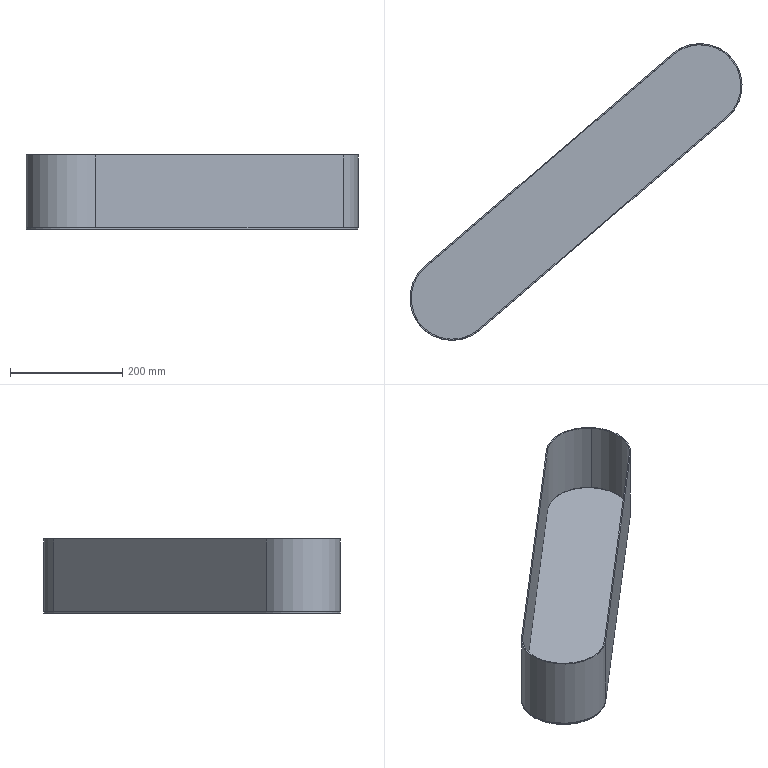Component | SolidWorks | BeltGuard-1 | 2 solids | 19 faces | box 591.77 x 528.9 x 132 mm | volume 633471 mm3 | plane 10 | cylinder 9 | commonest cylinder face diameters 150 x6 146 x3 | material Stainless Steel
build123d program:
from build123d import *

# Parameters (mm, degrees)
BOSS_EXTRUDE1_DEPTH = 2
BOSS_EXTRUDE2_DEPTH = 130


with BuildPart() as part:
    # Sketch1 → Boss-Extrude1 (new body)
    with BuildSketch(Plane.XY):
        with BuildLine():
            Line((0, 75), (582, 75))
            ThreePointArc((582, 75), (657, 0), (582, -75))
            Line((582, -75), (0, -75))
            ThreePointArc((0, -75), (-75, 0), (0, 75))
        make_face()
    extrude(amount=BOSS_EXTRUDE1_DEPTH)


with BuildPart() as body_2:
    # Sketch2 → Boss-Extrude2 (new body)
    with BuildSketch(Plane(origin=(0, 0, 0), x_dir=(-1, 0, 0), z_dir=(0, 0, -1))):
        with BuildLine():
            Line((0, 75), (-582, 75))
            ThreePointArc((-582, 75), (-657, 0), (-582, -75))
            Line((-582, -75), (0, -75))
            ThreePointArc((0, -75), (75, 0), (0, 75))
        make_face()
        with BuildLine():
            Line((0, 73), (-582, 73))
            ThreePointArc((-582, 73), (-655, 0), (-582, -73))
            Line((-582, -73), (0, -73))
            ThreePointArc((0, -73), (73, 0), (0, 73))
        make_face(mode=Mode.SUBTRACT)
    extrude(amount=BOSS_EXTRUDE2_DEPTH)


solid = Compound([part.part, body_2.part])

# Placed as in the assembly
solid = solid.moved(Location((-814.935, 937.863, -24.3), (180, 0, -40.619)))
STEP:
#1=COLOUR_RGB('',0.7922,0.8196,0.9333);
#2=FILL_AREA_STYLE_COLOUR('',#1);
#3=FILL_AREA_STYLE('',(#2));
#4=SURFACE_STYLE_FILL_AREA(#3);
#5=SURFACE_SIDE_STYLE('',(#4));
#6=SURFACE_STYLE_USAGE(.BOTH.,#5);
#7=PRESENTATION_STYLE_ASSIGNMENT((#6));
#8=CARTESIAN_POINT('',(-34.325,35.001,-1.035));
#9=VERTEX_POINT('',#8);
#10=CARTESIAN_POINT('',(-34.006,39.165,-1.035));
#11=VERTEX_POINT('',#10);
#12=CARTESIAN_POINT('',(-32.084,36.924,-1.035));
#13=DIRECTION('',(0.,0.,-1.));
#14=DIRECTION('',(0.7591,0.651,0.));
#15=AXIS2_PLACEMENT_3D('',#12,#13,#14);
#16=CIRCLE('',#15,2.953);
#17=EDGE_CURVE('',#9,#11,#16,.T.);
#18=ORIENTED_EDGE('',*,*,#17,.F.);
#19=CARTESIAN_POINT('',(-34.325,35.001,-0.9567));
#20=VERTEX_POINT('',#19);
#21=CARTESIAN_POINT('',(-34.325,35.001,-1.035));
#22=DIRECTION('',(-0.,-0.,1.));
#23=VECTOR('',#22,39.37);
#24=LINE('',#21,#23);
#25=EDGE_CURVE('',#9,#20,#24,.T.);
#26=ORIENTED_EDGE('',*,*,#25,.T.);
#27=CARTESIAN_POINT('',(-34.006,39.165,-0.9567));
#28=VERTEX_POINT('',#27);
#29=CARTESIAN_POINT('',(-32.084,36.924,-0.9567));
#30=DIRECTION('',(0.,0.,-1.));
#31=DIRECTION('',(0.7591,0.651,0.));
#32=AXIS2_PLACEMENT_3D('',#29,#30,#31);
#33=CIRCLE('',#32,2.953);
#34=EDGE_CURVE('',#20,#28,#33,.T.);
#35=ORIENTED_EDGE('',*,*,#34,.T.);
#36=CARTESIAN_POINT('',(-34.006,39.165,-1.035));
#37=DIRECTION('',(-0.,-0.,1.));
#38=VECTOR('',#37,39.37);
#39=LINE('',#36,#38);
#40=EDGE_CURVE('',#11,#28,#39,.T.);
#41=ORIENTED_EDGE('',*,*,#40,.F.);
#42=EDGE_LOOP('',(#18,#26,#35,#41));
#43=FACE_OUTER_BOUND('',#42,.T.);
#44=CARTESIAN_POINT('',(-32.084,36.924,-1.035));
#45=DIRECTION('',(-0.,-0.,1.));
#46=DIRECTION('',(-0.7591,-0.651,-0.));
#47=AXIS2_PLACEMENT_3D('',#44,#45,#46);
#48=CYLINDRICAL_SURFACE('',#47,2.953);
#49=ADVANCED_FACE('',(#43),#48,.T.);
#50=ORIENTED_EDGE('',*,*,#25,.F.);
#51=CARTESIAN_POINT('',(-30.162,34.682,-1.035));
#52=VERTEX_POINT('',#51);
#53=CARTESIAN_POINT('',(-32.084,36.924,-1.035));
#54=DIRECTION('',(0.,0.,-1.));
#55=DIRECTION('',(0.7591,0.651,0.));
#56=AXIS2_PLACEMENT_3D('',#53,#54,#55);
#57=CIRCLE('',#56,2.953);
#58=EDGE_CURVE('',#52,#9,#57,.T.);
#59=ORIENTED_EDGE('',*,*,#58,.F.);
#60=CARTESIAN_POINT('',(-30.162,34.682,-0.9567));
#61=VERTEX_POINT('',#60);
#62=CARTESIAN_POINT('',(-30.162,34.682,-1.035));
#63=DIRECTION('',(-0.,-0.,1.));
#64=VECTOR('',#63,39.37);
#65=LINE('',#62,#64);
#66=EDGE_CURVE('',#52,#61,#65,.T.);
#67=ORIENTED_EDGE('',*,*,#66,.T.);
#68=CARTESIAN_POINT('',(-32.084,36.924,-0.9567));
#69=DIRECTION('',(0.,0.,-1.));
#70=DIRECTION('',(0.7591,0.651,0.));
#71=AXIS2_PLACEMENT_3D('',#68,#69,#70);
#72=CIRCLE('',#71,2.953);
#73=EDGE_CURVE('',#61,#20,#72,.T.);
#74=ORIENTED_EDGE('',*,*,#73,.T.);
#75=EDGE_LOOP('',(#50,#59,#67,#74));
#76=FACE_OUTER_BOUND('',#75,.T.);
#77=CARTESIAN_POINT('',(-32.084,36.924,-1.035));
#78=DIRECTION('',(-0.,-0.,1.));
#79=DIRECTION('',(-0.7591,-0.651,-0.));
#80=AXIS2_PLACEMENT_3D('',#77,#78,#79);
#81=CYLINDRICAL_SURFACE('',#80,2.953);
#82=ADVANCED_FACE('',(#76),#81,.T.);
#83=CARTESIAN_POINT('',(-16.614,54.082,-0.9567));
#84=VERTEX_POINT('',#83);
#85=CARTESIAN_POINT('',(-34.006,39.165,-0.9567));
#86=DIRECTION('',(0.7591,0.651,0.));
#87=VECTOR('',#86,39.37);
#88=LINE('',#85,#87);
#89=EDGE_CURVE('',#28,#84,#88,.T.);
#90=ORIENTED_EDGE('',*,*,#89,.T.);
#91=CARTESIAN_POINT('',(-16.614,54.082,-1.035));
#92=VERTEX_POINT('',#91);
#93=CARTESIAN_POINT('',(-16.614,54.082,-1.035));
#94=DIRECTION('',(-0.,-0.,1.));
#95=VECTOR('',#94,39.37);
#96=LINE('',#93,#95);
#97=EDGE_CURVE('',#92,#84,#96,.T.);
#98=ORIENTED_EDGE('',*,*,#97,.F.);
#99=CARTESIAN_POINT('',(-34.006,39.165,-1.035));
#100=DIRECTION('',(0.7591,0.651,0.));
#101=VECTOR('',#100,39.37);
#102=LINE('',#99,#101);
#103=EDGE_CURVE('',#11,#92,#102,.T.);
#104=ORIENTED_EDGE('',*,*,#103,.F.);
#105=ORIENTED_EDGE('',*,*,#40,.T.);
#106=EDGE_LOOP('',(#90,#98,#104,#105));
#107=FACE_OUTER_BOUND('',#106,.T.);
#108=CARTESIAN_POINT('',(-34.006,39.165,-1.035));
#109=DIRECTION('',(0.651,-0.7591,-0.));
#110=DIRECTION('',(-0.7591,-0.651,-0.));
#111=AXIS2_PLACEMENT_3D('',#108,#109,#110);
#112=PLANE('',#111);
#113=ADVANCED_FACE('',(#107),#112,.F.);
#114=CARTESIAN_POINT('',(-12.769,49.6,-0.9567));
#115=VERTEX_POINT('',#114);
#116=CARTESIAN_POINT('',(-14.692,51.841,-0.9567));
#117=DIRECTION('',(0.,0.,-1.));
#118=DIRECTION('',(0.7591,0.651,0.));
#119=AXIS2_PLACEMENT_3D('',#116,#117,#118);
#120=CIRCLE('',#119,2.953);
#121=EDGE_CURVE('',#84,#115,#120,.T.);
#122=ORIENTED_EDGE('',*,*,#121,.T.);
#123=CARTESIAN_POINT('',(-12.769,49.6,-1.035));
#124=VERTEX_POINT('',#123);
#125=CARTESIAN_POINT('',(-12.769,49.6,-1.035));
#126=DIRECTION('',(-0.,-0.,1.));
#127=VECTOR('',#126,39.37);
#128=LINE('',#125,#127);
#129=EDGE_CURVE('',#124,#115,#128,.T.);
#130=ORIENTED_EDGE('',*,*,#129,.F.);
#131=CARTESIAN_POINT('',(-14.692,51.841,-1.035));
#132=DIRECTION('',(0.,0.,-1.));
#133=DIRECTION('',(0.7591,0.651,0.));
#134=AXIS2_PLACEMENT_3D('',#131,#132,#133);
#135=CIRCLE('',#134,2.953);
#136=EDGE_CURVE('',#92,#124,#135,.T.);
#137=ORIENTED_EDGE('',*,*,#136,.F.);
#138=ORIENTED_EDGE('',*,*,#97,.T.);
#139=EDGE_LOOP('',(#122,#130,#137,#138));
#140=FACE_OUTER_BOUND('',#139,.T.);
#141=CARTESIAN_POINT('',(-14.692,51.841,-1.035));
#142=DIRECTION('',(-0.,-0.,1.));
#143=DIRECTION('',(-0.7591,-0.651,-0.));
#144=AXIS2_PLACEMENT_3D('',#141,#142,#143);
#145=CYLINDRICAL_SURFACE('',#144,2.953);
#146=ADVANCED_FACE('',(#140),#145,.T.);
#147=CARTESIAN_POINT('',(-30.162,34.682,-0.9567));
#148=DIRECTION('',(-0.7591,-0.651,-0.));
#149=VECTOR('',#148,39.37);
#150=LINE('',#147,#149);
#151=EDGE_CURVE('',#115,#61,#150,.T.);
#152=ORIENTED_EDGE('',*,*,#151,.T.);
#153=ORIENTED_EDGE('',*,*,#66,.F.);
#154=CARTESIAN_POINT('',(-30.162,34.682,-1.035));
#155=DIRECTION('',(-0.7591,-0.651,-0.));
#156=VECTOR('',#155,39.37);
#157=LINE('',#154,#156);
#158=EDGE_CURVE('',#124,#52,#157,.T.);
#159=ORIENTED_EDGE('',*,*,#158,.F.);
#160=ORIENTED_EDGE('',*,*,#129,.T.);
#161=EDGE_LOOP('',(#152,#153,#159,#160));
#162=FACE_OUTER_BOUND('',#161,.T.);
#163=CARTESIAN_POINT('',(-30.162,34.682,-1.035));
#164=DIRECTION('',(-0.651,0.7591,0.));
#165=DIRECTION('',(0.7591,0.651,0.));
#166=AXIS2_PLACEMENT_3D('',#163,#164,#165);
#167=PLANE('',#166);
#168=ADVANCED_FACE('',(#162),#167,.F.);
#169=ORIENTED_EDGE('',*,*,#58,.T.);
#170=ORIENTED_EDGE('',*,*,#17,.T.);
#171=ORIENTED_EDGE('',*,*,#103,.T.);
#172=ORIENTED_EDGE('',*,*,#136,.T.);
#173=ORIENTED_EDGE('',*,*,#158,.T.);
#174=EDGE_LOOP('',(#169,#170,#171,#172,#173));
#175=FACE_OUTER_BOUND('',#174,.T.);
#176=CARTESIAN_POINT('',(-32.084,36.924,-1.035));
#177=DIRECTION('',(0.,0.,-1.));
#178=DIRECTION('',(0.7591,0.651,0.));
#179=AXIS2_PLACEMENT_3D('',#176,#177,#178);
#180=PLANE('',#179);
#181=ADVANCED_FACE('',(#175),#180,.T.);
#182=ORIENTED_EDGE('',*,*,#73,.F.);
#183=ORIENTED_EDGE('',*,*,#151,.F.);
#184=ORIENTED_EDGE('',*,*,#121,.F.);
#185=ORIENTED_EDGE('',*,*,#89,.F.);
#186=ORIENTED_EDGE('',*,*,#34,.F.);
#187=EDGE_LOOP('',(#182,#183,#184,#185,#186));
#188=FACE_OUTER_BOUND('',#187,.T.);
#189=CARTESIAN_POINT('',(-32.084,36.924,-0.9567));
#190=DIRECTION('',(0.,0.,-1.));
#191=DIRECTION('',(0.7591,0.651,0.));
#192=AXIS2_PLACEMENT_3D('',#189,#190,#191);
#193=PLANE('',#192);
#194=ADVANCED_FACE('',(#188),#193,.F.);
#195=CLOSED_SHELL('',(#49,#82,#113,#146,#168,#181,#194));
#196=MANIFOLD_SOLID_BREP('',#195);
#197=STYLED_ITEM('',(#7),#196);
#198=PRESENTATION_LAYER_ASSIGNMENT('','',(#197));
#199=CARTESIAN_POINT('',(-12.82,49.659,4.161));
#200=VERTEX_POINT('',#199);
#201=CARTESIAN_POINT('',(-12.51,53.712,4.161));
#202=VERTEX_POINT('',#201);
#203=CARTESIAN_POINT('',(-14.692,51.841,4.161));
#204=DIRECTION('',(-0.,-0.,1.));
#205=DIRECTION('',(-0.7591,-0.651,-0.));
#206=AXIS2_PLACEMENT_3D('',#203,#204,#205);
#207=CIRCLE('',#206,2.874);
#208=EDGE_CURVE('',#200,#202,#207,.T.);
#209=ORIENTED_EDGE('',*,*,#208,.T.);
#210=CARTESIAN_POINT('',(-12.51,53.712,-0.9567));
#211=VERTEX_POINT('',#210);
#212=CARTESIAN_POINT('',(-12.51,53.712,4.161));
#213=DIRECTION('',(0.,0.,-1.));
#214=VECTOR('',#213,39.37);
#215=LINE('',#212,#214);
#216=EDGE_CURVE('',#202,#211,#215,.T.);
#217=ORIENTED_EDGE('',*,*,#216,.T.);
#218=CARTESIAN_POINT('',(-12.82,49.659,-0.9567));
#219=VERTEX_POINT('',#218);
#220=CARTESIAN_POINT('',(-14.692,51.841,-0.9567));
#221=DIRECTION('',(-0.,-0.,1.));
#222=DIRECTION('',(-0.7591,-0.651,-0.));
#223=AXIS2_PLACEMENT_3D('',#220,#221,#222);
#224=CIRCLE('',#223,2.874);
#225=EDGE_CURVE('',#219,#211,#224,.T.);
#226=ORIENTED_EDGE('',*,*,#225,.F.);
#227=CARTESIAN_POINT('',(-12.82,49.659,4.161));
#228=DIRECTION('',(0.,0.,-1.));
#229=VECTOR('',#228,39.37);
#230=LINE('',#227,#229);
#231=EDGE_CURVE('',#200,#219,#230,.T.);
#232=ORIENTED_EDGE('',*,*,#231,.F.);
#233=EDGE_LOOP('',(#209,#217,#226,#232));
#234=FACE_OUTER_BOUND('',#233,.T.);
#235=CARTESIAN_POINT('',(-14.692,51.841,4.161));
#236=DIRECTION('',(0.,0.,-1.));
#237=DIRECTION('',(0.7591,0.651,0.));
#238=AXIS2_PLACEMENT_3D('',#235,#236,#237);
#239=CYLINDRICAL_SURFACE('',#238,2.874);
#240=ADVANCED_FACE('',(#234),#239,.F.);
#241=CARTESIAN_POINT('',(-12.45,53.763,4.161));
#242=VERTEX_POINT('',#241);
#243=CARTESIAN_POINT('',(-16.614,54.082,4.161));
#244=VERTEX_POINT('',#243);
#245=CARTESIAN_POINT('',(-14.692,51.841,4.161));
#246=DIRECTION('',(-0.,-0.,1.));
#247=DIRECTION('',(-0.7591,-0.651,-0.));
#248=AXIS2_PLACEMENT_3D('',#245,#246,#247);
#249=CIRCLE('',#248,2.953);
#250=EDGE_CURVE('',#242,#244,#249,.T.);
#251=ORIENTED_EDGE('',*,*,#250,.F.);
#252=CARTESIAN_POINT('',(-12.45,53.763,-0.9567));
#253=VERTEX_POINT('',#252);
#254=CARTESIAN_POINT('',(-12.45,53.763,4.161));
#255=DIRECTION('',(0.,0.,-1.));
#256=VECTOR('',#255,39.37);
#257=LINE('',#254,#256);
#258=EDGE_CURVE('',#242,#253,#257,.T.);
#259=ORIENTED_EDGE('',*,*,#258,.T.);
#260=CARTESIAN_POINT('',(-16.614,54.082,-0.9567));
#261=VERTEX_POINT('',#260);
#262=CARTESIAN_POINT('',(-14.692,51.841,-0.9567));
#263=DIRECTION('',(-0.,-0.,1.));
#264=DIRECTION('',(-0.7591,-0.651,-0.));
#265=AXIS2_PLACEMENT_3D('',#262,#263,#264);
#266=CIRCLE('',#265,2.953);
#267=EDGE_CURVE('',#253,#261,#266,.T.);
#268=ORIENTED_EDGE('',*,*,#267,.T.);
#269=CARTESIAN_POINT('',(-16.614,54.082,4.161));
#270=DIRECTION('',(0.,0.,-1.));
#271=VECTOR('',#270,39.37);
#272=LINE('',#269,#271);
#273=EDGE_CURVE('',#244,#261,#272,.T.);
#274=ORIENTED_EDGE('',*,*,#273,.F.);
#275=EDGE_LOOP('',(#251,#259,#268,#274));
#276=FACE_OUTER_BOUND('',#275,.T.);
#277=CARTESIAN_POINT('',(-14.692,51.841,4.161));
#278=DIRECTION('',(0.,0.,-1.));
#279=DIRECTION('',(0.7591,0.651,0.));
#280=AXIS2_PLACEMENT_3D('',#277,#278,#279);
#281=CYLINDRICAL_SURFACE('',#280,2.953);
#282=ADVANCED_FACE('',(#276),#281,.T.);
#283=CARTESIAN_POINT('',(-34.006,39.165,4.161));
#284=VERTEX_POINT('',#283);
#285=CARTESIAN_POINT('',(-30.162,34.682,4.161));
#286=VERTEX_POINT('',#285);
#287=CARTESIAN_POINT('',(-32.084,36.924,4.161));
#288=DIRECTION('',(-0.,-0.,1.));
#289=DIRECTION('',(-0.7591,-0.651,-0.));
#290=AXIS2_PLACEMENT_3D('',#287,#288,#289);
#291=CIRCLE('',#290,2.953);
#292=EDGE_CURVE('',#284,#286,#291,.T.);
#293=ORIENTED_EDGE('',*,*,#292,.T.);
#294=CARTESIAN_POINT('',(-12.769,49.6,4.161));
#295=VERTEX_POINT('',#294);
#296=CARTESIAN_POINT('',(-30.162,34.682,4.161));
#297=DIRECTION('',(0.7591,0.651,0.));
#298=VECTOR('',#297,39.37);
#299=LINE('',#296,#298);
#300=EDGE_CURVE('',#286,#295,#299,.T.);
#301=ORIENTED_EDGE('',*,*,#300,.T.);
#302=CARTESIAN_POINT('',(-14.692,51.841,4.161));
#303=DIRECTION('',(-0.,-0.,1.));
#304=DIRECTION('',(-0.7591,-0.651,-0.));
#305=AXIS2_PLACEMENT_3D('',#302,#303,#304);
#306=CIRCLE('',#305,2.953);
#307=EDGE_CURVE('',#295,#242,#306,.T.);
#308=ORIENTED_EDGE('',*,*,#307,.T.);
#309=ORIENTED_EDGE('',*,*,#250,.T.);
#310=CARTESIAN_POINT('',(-16.614,54.082,4.161));
#311=DIRECTION('',(-0.7591,-0.651,-0.));
#312=VECTOR('',#311,39.37);
#313=LINE('',#310,#312);
#314=EDGE_CURVE('',#244,#284,#313,.T.);
#315=ORIENTED_EDGE('',*,*,#314,.T.);
#316=EDGE_LOOP('',(#293,#301,#308,#309,#315));
#317=FACE_OUTER_BOUND('',#316,.T.);
#318=CARTESIAN_POINT('',(-30.213,34.742,4.161));
#319=VERTEX_POINT('',#318);
#320=CARTESIAN_POINT('',(-30.213,34.742,4.161));
#321=DIRECTION('',(0.7591,0.651,0.));
#322=VECTOR('',#321,39.37);
#323=LINE('',#320,#322);
#324=EDGE_CURVE('',#319,#200,#323,.T.);
#325=ORIENTED_EDGE('',*,*,#324,.F.);
#326=CARTESIAN_POINT('',(-33.955,39.105,4.161));
#327=VERTEX_POINT('',#326);
#328=CARTESIAN_POINT('',(-32.084,36.924,4.161));
#329=DIRECTION('',(-0.,-0.,1.));
#330=DIRECTION('',(-0.7591,-0.651,-0.));
#331=AXIS2_PLACEMENT_3D('',#328,#329,#330);
#332=CIRCLE('',#331,2.874);
#333=EDGE_CURVE('',#327,#319,#332,.T.);
#334=ORIENTED_EDGE('',*,*,#333,.F.);
#335=CARTESIAN_POINT('',(-16.563,54.023,4.161));
#336=VERTEX_POINT('',#335);
#337=CARTESIAN_POINT('',(-16.563,54.023,4.161));
#338=DIRECTION('',(-0.7591,-0.651,-0.));
#339=VECTOR('',#338,39.37);
#340=LINE('',#337,#339);
#341=EDGE_CURVE('',#336,#327,#340,.T.);
#342=ORIENTED_EDGE('',*,*,#341,.F.);
#343=CARTESIAN_POINT('',(-14.692,51.841,4.161));
#344=DIRECTION('',(-0.,-0.,1.));
#345=DIRECTION('',(-0.7591,-0.651,-0.));
#346=AXIS2_PLACEMENT_3D('',#343,#344,#345);
#347=CIRCLE('',#346,2.874);
#348=EDGE_CURVE('',#202,#336,#347,.T.);
#349=ORIENTED_EDGE('',*,*,#348,.F.);
#350=ORIENTED_EDGE('',*,*,#208,.F.);
#351=EDGE_LOOP('',(#325,#334,#342,#349,#350));
#352=FACE_BOUND('',#351,.T.);
#353=CARTESIAN_POINT('',(-32.084,36.924,4.161));
#354=DIRECTION('',(-0.,-0.,1.));
#355=DIRECTION('',(-0.7591,-0.651,-0.));
#356=AXIS2_PLACEMENT_3D('',#353,#354,#355);
#357=PLANE('',#356);
#358=ADVANCED_FACE('',(#317,#352),#357,.T.);
#359=CARTESIAN_POINT('',(-34.006,39.165,-0.9567));
#360=VERTEX_POINT('',#359);
#361=CARTESIAN_POINT('',(-30.162,34.682,-0.9567));
#362=VERTEX_POINT('',#361);
#363=CARTESIAN_POINT('',(-32.084,36.924,-0.9567));
#364=DIRECTION('',(-0.,-0.,1.));
#365=DIRECTION('',(-0.7591,-0.651,-0.));
#366=AXIS2_PLACEMENT_3D('',#363,#364,#365);
#367=CIRCLE('',#366,2.953);
#368=EDGE_CURVE('',#360,#362,#367,.T.);
#369=ORIENTED_EDGE('',*,*,#368,.F.);
#370=CARTESIAN_POINT('',(-16.614,54.082,-0.9567));
#371=DIRECTION('',(-0.7591,-0.651,-0.));
#372=VECTOR('',#371,39.37);
#373=LINE('',#370,#372);
#374=EDGE_CURVE('',#261,#360,#373,.T.);
#375=ORIENTED_EDGE('',*,*,#374,.F.);
#376=ORIENTED_EDGE('',*,*,#267,.F.);
#377=CARTESIAN_POINT('',(-12.769,49.6,-0.9567));
#378=VERTEX_POINT('',#377);
#379=CARTESIAN_POINT('',(-14.692,51.841,-0.9567));
#380=DIRECTION('',(-0.,-0.,1.));
#381=DIRECTION('',(-0.7591,-0.651,-0.));
#382=AXIS2_PLACEMENT_3D('',#379,#380,#381);
#383=CIRCLE('',#382,2.953);
#384=EDGE_CURVE('',#378,#253,#383,.T.);
#385=ORIENTED_EDGE('',*,*,#384,.F.);
#386=CARTESIAN_POINT('',(-30.162,34.682,-0.9567));
#387=DIRECTION('',(0.7591,0.651,0.));
#388=VECTOR('',#387,39.37);
#389=LINE('',#386,#388);
#390=EDGE_CURVE('',#362,#378,#389,.T.);
#391=ORIENTED_EDGE('',*,*,#390,.F.);
#392=EDGE_LOOP('',(#369,#375,#376,#385,#391));
#393=FACE_OUTER_BOUND('',#392,.T.);
#394=CARTESIAN_POINT('',(-33.955,39.105,-0.9567));
#395=VERTEX_POINT('',#394);
#396=CARTESIAN_POINT('',(-30.213,34.742,-0.9567));
#397=VERTEX_POINT('',#396);
#398=CARTESIAN_POINT('',(-32.084,36.924,-0.9567));
#399=DIRECTION('',(-0.,-0.,1.));
#400=DIRECTION('',(-0.7591,-0.651,-0.));
#401=AXIS2_PLACEMENT_3D('',#398,#399,#400);
#402=CIRCLE('',#401,2.874);
#403=EDGE_CURVE('',#395,#397,#402,.T.);
#404=ORIENTED_EDGE('',*,*,#403,.T.);
#405=CARTESIAN_POINT('',(-30.213,34.742,-0.9567));
#406=DIRECTION('',(0.7591,0.651,0.));
#407=VECTOR('',#406,39.37);
#408=LINE('',#405,#407);
#409=EDGE_CURVE('',#397,#219,#408,.T.);
#410=ORIENTED_EDGE('',*,*,#409,.T.);
#411=ORIENTED_EDGE('',*,*,#225,.T.);
#412=CARTESIAN_POINT('',(-16.563,54.023,-0.9567));
#413=VERTEX_POINT('',#412);
#414=CARTESIAN_POINT('',(-14.692,51.841,-0.9567));
#415=DIRECTION('',(-0.,-0.,1.));
#416=DIRECTION('',(-0.7591,-0.651,-0.));
#417=AXIS2_PLACEMENT_3D('',#414,#415,#416);
#418=CIRCLE('',#417,2.874);
#419=EDGE_CURVE('',#211,#413,#418,.T.);
#420=ORIENTED_EDGE('',*,*,#419,.T.);
#421=CARTESIAN_POINT('',(-16.563,54.023,-0.9567));
#422=DIRECTION('',(-0.7591,-0.651,-0.));
#423=VECTOR('',#422,39.37);
#424=LINE('',#421,#423);
#425=EDGE_CURVE('',#413,#395,#424,.T.);
#426=ORIENTED_EDGE('',*,*,#425,.T.);
#427=EDGE_LOOP('',(#404,#410,#411,#420,#426));
#428=FACE_BOUND('',#427,.T.);
#429=CARTESIAN_POINT('',(-32.084,36.924,-0.9567));
#430=DIRECTION('',(-0.,-0.,1.));
#431=DIRECTION('',(-0.7591,-0.651,-0.));
#432=AXIS2_PLACEMENT_3D('',#429,#430,#431);
#433=PLANE('',#432);
#434=ADVANCED_FACE('',(#393,#428),#433,.F.);
#435=ORIENTED_EDGE('',*,*,#368,.T.);
#436=CARTESIAN_POINT('',(-30.162,34.682,4.161));
#437=DIRECTION('',(0.,0.,-1.));
#438=VECTOR('',#437,39.37);
#439=LINE('',#436,#438);
#440=EDGE_CURVE('',#286,#362,#439,.T.);
#441=ORIENTED_EDGE('',*,*,#440,.F.);
#442=ORIENTED_EDGE('',*,*,#292,.F.);
#443=CARTESIAN_POINT('',(-34.006,39.165,4.161));
#444=DIRECTION('',(0.,0.,-1.));
#445=VECTOR('',#444,39.37);
#446=LINE('',#443,#445);
#447=EDGE_CURVE('',#284,#360,#446,.T.);
#448=ORIENTED_EDGE('',*,*,#447,.T.);
#449=EDGE_LOOP('',(#435,#441,#442,#448));
#450=FACE_OUTER_BOUND('',#449,.T.);
#451=CARTESIAN_POINT('',(-32.084,36.924,4.161));
#452=DIRECTION('',(0.,0.,-1.));
#453=DIRECTION('',(0.7591,0.651,0.));
#454=AXIS2_PLACEMENT_3D('',#451,#452,#453);
#455=CYLINDRICAL_SURFACE('',#454,2.953);
#456=ADVANCED_FACE('',(#450),#455,.T.);
#457=ORIENTED_EDGE('',*,*,#390,.T.);
#458=CARTESIAN_POINT('',(-12.769,49.6,4.161));
#459=DIRECTION('',(0.,0.,-1.));
#460=VECTOR('',#459,39.37);
#461=LINE('',#458,#460);
#462=EDGE_CURVE('',#295,#378,#461,.T.);
#463=ORIENTED_EDGE('',*,*,#462,.F.);
#464=ORIENTED_EDGE('',*,*,#300,.F.);
#465=ORIENTED_EDGE('',*,*,#440,.T.);
#466=EDGE_LOOP('',(#457,#463,#464,#465));
#467=FACE_OUTER_BOUND('',#466,.T.);
#468=CARTESIAN_POINT('',(-30.162,34.682,4.161));
#469=DIRECTION('',(-0.651,0.7591,0.));
#470=DIRECTION('',(0.7591,0.651,0.));
#471=AXIS2_PLACEMENT_3D('',#468,#469,#470);
#472=PLANE('',#471);
#473=ADVANCED_FACE('',(#467),#472,.F.);
#474=ORIENTED_EDGE('',*,*,#258,.F.);
#475=ORIENTED_EDGE('',*,*,#307,.F.);
#476=ORIENTED_EDGE('',*,*,#462,.T.);
#477=ORIENTED_EDGE('',*,*,#384,.T.);
#478=EDGE_LOOP('',(#474,#475,#476,#477));
#479=FACE_OUTER_BOUND('',#478,.T.);
#480=CARTESIAN_POINT('',(-14.692,51.841,4.161));
#481=DIRECTION('',(0.,0.,-1.));
#482=DIRECTION('',(0.7591,0.651,0.));
#483=AXIS2_PLACEMENT_3D('',#480,#481,#482);
#484=CYLINDRICAL_SURFACE('',#483,2.953);
#485=ADVANCED_FACE('',(#479),#484,.T.);
#486=ORIENTED_EDGE('',*,*,#374,.T.);
#487=ORIENTED_EDGE('',*,*,#447,.F.);
#488=ORIENTED_EDGE('',*,*,#314,.F.);
#489=ORIENTED_EDGE('',*,*,#273,.T.);
#490=EDGE_LOOP('',(#486,#487,#488,#489));
#491=FACE_OUTER_BOUND('',#490,.T.);
#492=CARTESIAN_POINT('',(-16.614,54.082,4.161));
#493=DIRECTION('',(0.651,-0.7591,-0.));
#494=DIRECTION('',(-0.7591,-0.651,-0.));
#495=AXIS2_PLACEMENT_3D('',#492,#493,#494);
#496=PLANE('',#495);
#497=ADVANCED_FACE('',(#491),#496,.F.);
#498=ORIENTED_EDGE('',*,*,#403,.F.);
#499=CARTESIAN_POINT('',(-33.955,39.105,4.161));
#500=DIRECTION('',(0.,0.,-1.));
#501=VECTOR('',#500,39.37);
#502=LINE('',#499,#501);
#503=EDGE_CURVE('',#327,#395,#502,.T.);
#504=ORIENTED_EDGE('',*,*,#503,.F.);
#505=ORIENTED_EDGE('',*,*,#333,.T.);
#506=CARTESIAN_POINT('',(-30.213,34.742,4.161));
#507=DIRECTION('',(0.,0.,-1.));
#508=VECTOR('',#507,39.37);
#509=LINE('',#506,#508);
#510=EDGE_CURVE('',#319,#397,#509,.T.);
#511=ORIENTED_EDGE('',*,*,#510,.T.);
#512=EDGE_LOOP('',(#498,#504,#505,#511));
#513=FACE_OUTER_BOUND('',#512,.T.);
#514=CARTESIAN_POINT('',(-32.084,36.924,4.161));
#515=DIRECTION('',(0.,0.,-1.));
#516=DIRECTION('',(0.7591,0.651,0.));
#517=AXIS2_PLACEMENT_3D('',#514,#515,#516);
#518=CYLINDRICAL_SURFACE('',#517,2.874);
#519=ADVANCED_FACE('',(#513),#518,.F.);
#520=ORIENTED_EDGE('',*,*,#409,.F.);
#521=ORIENTED_EDGE('',*,*,#510,.F.);
#522=ORIENTED_EDGE('',*,*,#324,.T.);
#523=ORIENTED_EDGE('',*,*,#231,.T.);
#524=EDGE_LOOP('',(#520,#521,#522,#523));
#525=FACE_OUTER_BOUND('',#524,.T.);
#526=CARTESIAN_POINT('',(-30.213,34.742,4.161));
#527=DIRECTION('',(-0.651,0.7591,0.));
#528=DIRECTION('',(0.7591,0.651,0.));
#529=AXIS2_PLACEMENT_3D('',#526,#527,#528);
#530=PLANE('',#529);
#531=ADVANCED_FACE('',(#525),#530,.T.);
#532=ORIENTED_EDGE('',*,*,#216,.F.);
#533=ORIENTED_EDGE('',*,*,#348,.T.);
#534=CARTESIAN_POINT('',(-16.563,54.023,4.161));
#535=DIRECTION('',(0.,0.,-1.));
#536=VECTOR('',#535,39.37);
#537=LINE('',#534,#536);
#538=EDGE_CURVE('',#336,#413,#537,.T.);
#539=ORIENTED_EDGE('',*,*,#538,.T.);
#540=ORIENTED_EDGE('',*,*,#419,.F.);
#541=EDGE_LOOP('',(#532,#533,#539,#540));
#542=FACE_OUTER_BOUND('',#541,.T.);
#543=CARTESIAN_POINT('',(-14.692,51.841,4.161));
#544=DIRECTION('',(0.,0.,-1.));
#545=DIRECTION('',(0.7591,0.651,0.));
#546=AXIS2_PLACEMENT_3D('',#543,#544,#545);
#547=CYLINDRICAL_SURFACE('',#546,2.874);
#548=ADVANCED_FACE('',(#542),#547,.F.);
#549=ORIENTED_EDGE('',*,*,#425,.F.);
#550=ORIENTED_EDGE('',*,*,#538,.F.);
#551=ORIENTED_EDGE('',*,*,#341,.T.);
#552=ORIENTED_EDGE('',*,*,#503,.T.);
#553=EDGE_LOOP('',(#549,#550,#551,#552));
#554=FACE_OUTER_BOUND('',#553,.T.);
#555=CARTESIAN_POINT('',(-16.563,54.023,4.161));
#556=DIRECTION('',(0.651,-0.7591,-0.));
#557=DIRECTION('',(-0.7591,-0.651,-0.));
#558=AXIS2_PLACEMENT_3D('',#555,#556,#557);
#559=PLANE('',#558);
#560=ADVANCED_FACE('',(#554),#559,.T.);
#561=CLOSED_SHELL('',(#240,#282,#358,#434,#456,#473,#485,#497,#519,#531,#548,#560));
#562=MANIFOLD_SOLID_BREP('',#561);
#563=CARTESIAN_POINT('',(0.,0.,0.));
#564=DIRECTION('',(0.,0.,1.));
#565=DIRECTION('',(1.,0.,0.));
#566=AXIS2_PLACEMENT_3D('',#563,#564,#565);
#567=(LENGTH_UNIT()NAMED_UNIT(*)SI_UNIT($,.METRE.));
#568=LENGTH_MEASURE_WITH_UNIT(LENGTH_MEASURE(0.0254),#567);
#569=DIMENSIONAL_EXPONENTS(1.,0.,0.,0.,0.,0.,0.);
#570=(CONVERSION_BASED_UNIT('',#568)LENGTH_UNIT()NAMED_UNIT(#569));
#571=UNCERTAINTY_MEASURE_WITH_UNIT(LENGTH_MEASURE(0.00001),#570,'','');
#572=(NAMED_UNIT(*)PLANE_ANGLE_UNIT()SI_UNIT($,.RADIAN.));
#573=(NAMED_UNIT(*)SI_UNIT($,.STERADIAN.)SOLID_ANGLE_UNIT());
#574=(GEOMETRIC_REPRESENTATION_CONTEXT(3)GLOBAL_UNCERTAINTY_ASSIGNED_CONTEXT((#571))GLOBAL_UNIT_ASSIGNED_CONTEXT((#570,#572,#573))REPRESENTATION_CONTEXT('',''));
#575=ADVANCED_BREP_SHAPE_REPRESENTATION('',(#562,#196,#566),#574);
#576=(LENGTH_UNIT()NAMED_UNIT(*)SI_UNIT($,.METRE.));
#577=LENGTH_MEASURE_WITH_UNIT(LENGTH_MEASURE(0.0254),#576);
#578=DIMENSIONAL_EXPONENTS(1.,0.,0.,0.,0.,0.,0.);
#579=(CONVERSION_BASED_UNIT('',#577)LENGTH_UNIT()NAMED_UNIT(#578));
#580=UNCERTAINTY_MEASURE_WITH_UNIT(LENGTH_MEASURE(0.00001),#579,'','');
#581=(NAMED_UNIT(*)PLANE_ANGLE_UNIT()SI_UNIT($,.RADIAN.));
#582=(NAMED_UNIT(*)SI_UNIT($,.STERADIAN.)SOLID_ANGLE_UNIT());
#583=(GEOMETRIC_REPRESENTATION_CONTEXT(3)GLOBAL_UNCERTAINTY_ASSIGNED_CONTEXT((#580))GLOBAL_UNIT_ASSIGNED_CONTEXT((#579,#581,#582))REPRESENTATION_CONTEXT('',''));
#584=MECHANICAL_DESIGN_GEOMETRIC_PRESENTATION_REPRESENTATION('',(#197),#583);
#585=COLOUR_RGB('',0.7922,0.8196,0.9333);
#586=FILL_AREA_STYLE_COLOUR('',#585);
#587=FILL_AREA_STYLE('',(#586));
#588=SURFACE_STYLE_FILL_AREA(#587);
#589=SURFACE_SIDE_STYLE('',(#588));
#590=SURFACE_STYLE_USAGE(.BOTH.,#589);
#591=PRESENTATION_STYLE_ASSIGNMENT((#590));
#592=STYLED_ITEM('',(#591),#562);
#593=PRESENTATION_LAYER_ASSIGNMENT('','',(#592));
#594=(LENGTH_UNIT()NAMED_UNIT(*)SI_UNIT($,.METRE.));
#595=LENGTH_MEASURE_WITH_UNIT(LENGTH_MEASURE(0.0254),#594);
#596=DIMENSIONAL_EXPONENTS(1.,0.,0.,0.,0.,0.,0.);
#597=(CONVERSION_BASED_UNIT('',#595)LENGTH_UNIT()NAMED_UNIT(#596));
#598=UNCERTAINTY_MEASURE_WITH_UNIT(LENGTH_MEASURE(0.00001),#597,'','');
#599=(NAMED_UNIT(*)PLANE_ANGLE_UNIT()SI_UNIT($,.RADIAN.));
#600=(NAMED_UNIT(*)SI_UNIT($,.STERADIAN.)SOLID_ANGLE_UNIT());
#601=(GEOMETRIC_REPRESENTATION_CONTEXT(3)GLOBAL_UNCERTAINTY_ASSIGNED_CONTEXT((#598))GLOBAL_UNIT_ASSIGNED_CONTEXT((#597,#599,#600))REPRESENTATION_CONTEXT('',''));
#602=MECHANICAL_DESIGN_GEOMETRIC_PRESENTATION_REPRESENTATION('',(#592),#601);